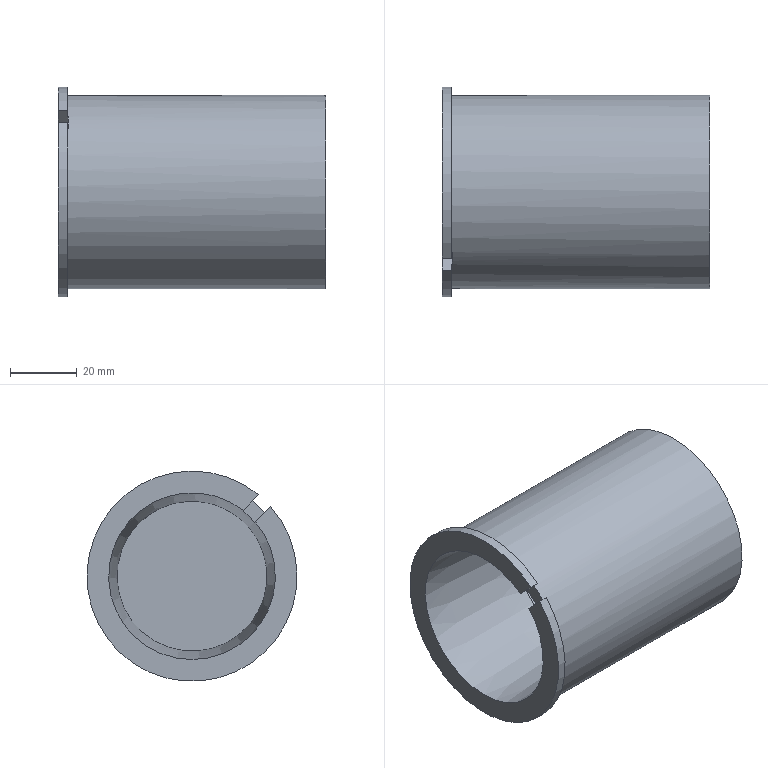Component | NX | SIM15_C1_ACHSE | 1 solid | 12 faces | volume 143224 mm3 | plane 7 | cylinder 3 | cone 2 | commonest cylinder face diameters 58 x1 63 x1 45 x1